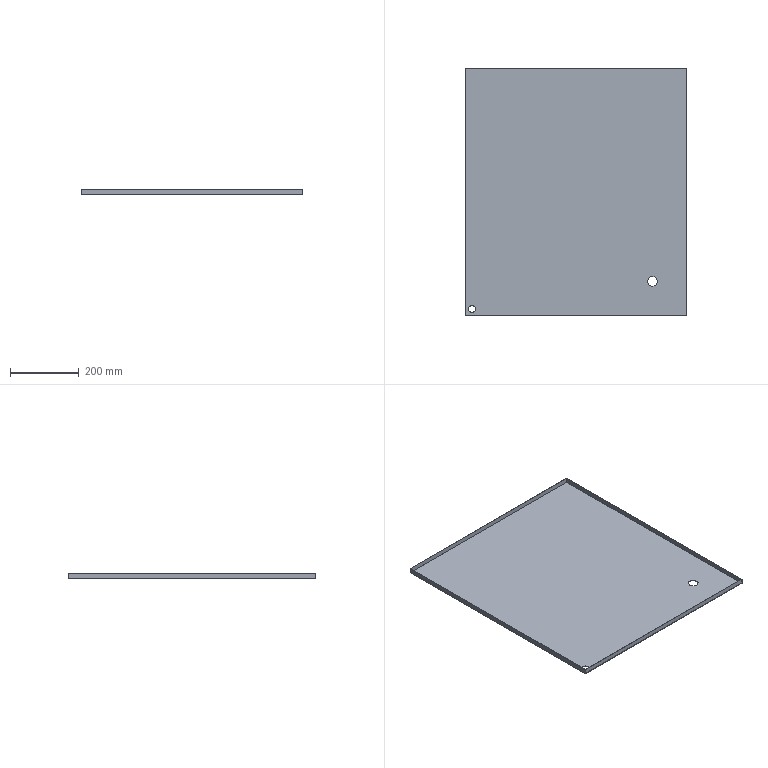Component | SolidWorks | FrameAssembly-1_FrameWeldment-1_RearThinPlate-1 | 1 solid | 15 faces | box 643 x 718 x 15 mm | volume 597890 mm3 | plane 11 | cylinder 4 | commonest cylinder face diameters 20 x2 28 x2
build123d program:
from build123d import *

# Parameters (mm, degrees)
SKETCH1_W                      = 643
SKETCH1_H                      = 718
BOSS_EXTRUDE1_DEPTH            = 15
SKETCH2_W                      = 640.6
SKETCH2_H                      = 715.6
CUT_EXTRUDE1_DEPTH             = 13.8
M24_CLEARANCE_HOLE_1_D         = 28
M24_CLEARANCE_HOLE_1_DEPTH     = 15
F_20_0_20_DIAMETER_HOLE1_D     = 20
F_20_0_20_DIAMETER_HOLE1_DEPTH = 15


with BuildPart() as part:
    # Sketch1 → Boss-Extrude1 (new body)
    with BuildSketch(Plane(origin=(0, 0, 0), x_dir=(-1, 0, 0), z_dir=(0, 0, -1))):
        Rectangle(SKETCH1_W, SKETCH1_H)
    extrude(amount=-BOSS_EXTRUDE1_DEPTH)

    # Sketch2 → Cut-Extrude1 (cut)
    with BuildSketch(Plane(origin=(0, 0, 0), x_dir=(-1, 0, 0), z_dir=(0, 0, -1))):
        Rectangle(SKETCH2_W, SKETCH2_H)
    extrude(amount=-CUT_EXTRUDE1_DEPTH, mode=Mode.SUBTRACT)

    # M24 Clearance Hole 1
    with Locations(Plane.XY.offset(15)):
        with Locations((-221.5, -259)):
            Hole(M24_CLEARANCE_HOLE_1_D / 2, depth=M24_CLEARANCE_HOLE_1_DEPTH)

    # 20.0 _20_ Diameter Hole1
    with Locations(Plane.XY.offset(15)):
        with Locations((301.5, -339)):
            Hole(F_20_0_20_DIAMETER_HOLE1_D / 2, depth=F_20_0_20_DIAMETER_HOLE1_DEPTH)


solid = part.part

# Placed as in the assembly
solid = solid.moved(Location((-298.746, -38.627, -351.5), (-180, 0, 180)))
STEP:
#1=CARTESIAN_POINT('',(-24.025,-14.867,-14.382));
#2=VERTEX_POINT('',#1);
#3=CARTESIAN_POINT('',(-23.238,-14.867,-14.382));
#4=VERTEX_POINT('',#3);
#5=CARTESIAN_POINT('',(-23.632,-14.867,-14.382));
#6=DIRECTION('',(0.,0.,1.));
#7=DIRECTION('',(1.,0.,0.));
#8=AXIS2_PLACEMENT_3D('',#5,#6,#7);
#9=CIRCLE('',#8,0.3937);
#10=EDGE_CURVE('',#2,#4,#9,.T.);
#11=ORIENTED_EDGE('',*,*,#10,.T.);
#12=CARTESIAN_POINT('',(-23.238,-14.867,-14.429));
#13=VERTEX_POINT('',#12);
#14=CARTESIAN_POINT('',(-23.238,-14.867,-14.429));
#15=DIRECTION('',(-0.,-0.,-1.));
#16=VECTOR('',#15,39.37);
#17=LINE('',#14,#16);
#18=EDGE_CURVE('',#4,#13,#17,.T.);
#19=ORIENTED_EDGE('',*,*,#18,.T.);
#20=CARTESIAN_POINT('',(-24.025,-14.867,-14.429));
#21=VERTEX_POINT('',#20);
#22=CARTESIAN_POINT('',(-23.632,-14.867,-14.429));
#23=DIRECTION('',(-0.,-0.,-1.));
#24=DIRECTION('',(-1.,0.,0.));
#25=AXIS2_PLACEMENT_3D('',#22,#23,#24);
#26=CIRCLE('',#25,0.3937);
#27=EDGE_CURVE('',#13,#21,#26,.T.);
#28=ORIENTED_EDGE('',*,*,#27,.T.);
#29=CARTESIAN_POINT('',(-24.025,-14.867,-14.429));
#30=DIRECTION('',(-0.,-0.,-1.));
#31=VECTOR('',#30,39.37);
#32=LINE('',#29,#31);
#33=EDGE_CURVE('',#2,#21,#32,.T.);
#34=ORIENTED_EDGE('',*,*,#33,.F.);
#35=EDGE_LOOP('',(#11,#19,#28,#34));
#36=FACE_OUTER_BOUND('',#35,.T.);
#37=CARTESIAN_POINT('',(-23.632,-14.867,-14.429));
#38=DIRECTION('',(-0.,-0.,-1.));
#39=DIRECTION('',(-1.,0.,0.));
#40=AXIS2_PLACEMENT_3D('',#37,#38,#39);
#41=CYLINDRICAL_SURFACE('',#40,0.3937);
#42=ADVANCED_FACE('',(#36),#41,.F.);
#43=CARTESIAN_POINT('',(-3.592,-11.718,-14.382));
#44=VERTEX_POINT('',#43);
#45=CARTESIAN_POINT('',(-2.49,-11.718,-14.382));
#46=VERTEX_POINT('',#45);
#47=CARTESIAN_POINT('',(-3.041,-11.718,-14.382));
#48=DIRECTION('',(0.,0.,1.));
#49=DIRECTION('',(1.,0.,0.));
#50=AXIS2_PLACEMENT_3D('',#47,#48,#49);
#51=CIRCLE('',#50,0.5512);
#52=EDGE_CURVE('',#44,#46,#51,.T.);
#53=ORIENTED_EDGE('',*,*,#52,.T.);
#54=CARTESIAN_POINT('',(-2.49,-11.718,-14.429));
#55=VERTEX_POINT('',#54);
#56=CARTESIAN_POINT('',(-2.49,-11.718,-14.429));
#57=DIRECTION('',(-0.,-0.,-1.));
#58=VECTOR('',#57,39.37);
#59=LINE('',#56,#58);
#60=EDGE_CURVE('',#46,#55,#59,.T.);
#61=ORIENTED_EDGE('',*,*,#60,.T.);
#62=CARTESIAN_POINT('',(-3.592,-11.718,-14.429));
#63=VERTEX_POINT('',#62);
#64=CARTESIAN_POINT('',(-3.041,-11.718,-14.429));
#65=DIRECTION('',(-0.,-0.,-1.));
#66=DIRECTION('',(-1.,0.,0.));
#67=AXIS2_PLACEMENT_3D('',#64,#65,#66);
#68=CIRCLE('',#67,0.5512);
#69=EDGE_CURVE('',#55,#63,#68,.T.);
#70=ORIENTED_EDGE('',*,*,#69,.T.);
#71=CARTESIAN_POINT('',(-3.592,-11.718,-14.429));
#72=DIRECTION('',(-0.,-0.,-1.));
#73=VECTOR('',#72,39.37);
#74=LINE('',#71,#73);
#75=EDGE_CURVE('',#44,#63,#74,.T.);
#76=ORIENTED_EDGE('',*,*,#75,.F.);
#77=EDGE_LOOP('',(#53,#61,#70,#76));
#78=FACE_OUTER_BOUND('',#77,.T.);
#79=CARTESIAN_POINT('',(-3.041,-11.718,-14.429));
#80=DIRECTION('',(-0.,-0.,-1.));
#81=DIRECTION('',(-1.,0.,0.));
#82=AXIS2_PLACEMENT_3D('',#79,#80,#81);
#83=CYLINDRICAL_SURFACE('',#82,0.5512);
#84=ADVANCED_FACE('',(#78),#83,.F.);
#85=CARTESIAN_POINT('',(-24.419,-15.655,-13.839));
#86=VERTEX_POINT('',#85);
#87=CARTESIAN_POINT('',(0.8958,-15.655,-13.839));
#88=VERTEX_POINT('',#87);
#89=CARTESIAN_POINT('',(-24.419,-15.655,-13.839));
#90=DIRECTION('',(1.,0.,-0.));
#91=VECTOR('',#90,39.37);
#92=LINE('',#89,#91);
#93=EDGE_CURVE('',#86,#88,#92,.T.);
#94=ORIENTED_EDGE('',*,*,#93,.F.);
#95=CARTESIAN_POINT('',(-24.419,-15.655,-14.429));
#96=VERTEX_POINT('',#95);
#97=CARTESIAN_POINT('',(-24.419,-15.655,-14.429));
#98=DIRECTION('',(0.,0.,1.));
#99=VECTOR('',#98,39.37);
#100=LINE('',#97,#99);
#101=EDGE_CURVE('',#96,#86,#100,.T.);
#102=ORIENTED_EDGE('',*,*,#101,.F.);
#103=CARTESIAN_POINT('',(0.8958,-15.655,-14.429));
#104=VERTEX_POINT('',#103);
#105=CARTESIAN_POINT('',(-24.419,-15.655,-14.429));
#106=DIRECTION('',(1.,0.,-0.));
#107=VECTOR('',#106,39.37);
#108=LINE('',#105,#107);
#109=EDGE_CURVE('',#96,#104,#108,.T.);
#110=ORIENTED_EDGE('',*,*,#109,.T.);
#111=CARTESIAN_POINT('',(0.8958,-15.655,-14.429));
#112=DIRECTION('',(0.,0.,1.));
#113=VECTOR('',#112,39.37);
#114=LINE('',#111,#113);
#115=EDGE_CURVE('',#104,#88,#114,.T.);
#116=ORIENTED_EDGE('',*,*,#115,.T.);
#117=EDGE_LOOP('',(#94,#102,#110,#116));
#118=FACE_OUTER_BOUND('',#117,.T.);
#119=CARTESIAN_POINT('',(-24.419,-15.655,-14.429));
#120=DIRECTION('',(0.,-1.,0.));
#121=DIRECTION('',(0.,0.,1.));
#122=AXIS2_PLACEMENT_3D('',#119,#120,#121);
#123=PLANE('',#122);
#124=ADVANCED_FACE('',(#118),#123,.T.);
#125=CARTESIAN_POINT('',(-24.419,12.613,-13.839));
#126=VERTEX_POINT('',#125);
#127=CARTESIAN_POINT('',(-24.419,12.613,-13.839));
#128=DIRECTION('',(0.,-1.,0.));
#129=VECTOR('',#128,39.37);
#130=LINE('',#127,#129);
#131=EDGE_CURVE('',#126,#86,#130,.T.);
#132=ORIENTED_EDGE('',*,*,#131,.F.);
#133=CARTESIAN_POINT('',(-24.419,12.613,-14.429));
#134=VERTEX_POINT('',#133);
#135=CARTESIAN_POINT('',(-24.419,12.613,-14.429));
#136=DIRECTION('',(0.,0.,1.));
#137=VECTOR('',#136,39.37);
#138=LINE('',#135,#137);
#139=EDGE_CURVE('',#134,#126,#138,.T.);
#140=ORIENTED_EDGE('',*,*,#139,.F.);
#141=CARTESIAN_POINT('',(-24.419,12.613,-14.429));
#142=DIRECTION('',(0.,-1.,0.));
#143=VECTOR('',#142,39.37);
#144=LINE('',#141,#143);
#145=EDGE_CURVE('',#134,#96,#144,.T.);
#146=ORIENTED_EDGE('',*,*,#145,.T.);
#147=ORIENTED_EDGE('',*,*,#101,.T.);
#148=EDGE_LOOP('',(#132,#140,#146,#147));
#149=FACE_OUTER_BOUND('',#148,.T.);
#150=CARTESIAN_POINT('',(-24.419,12.613,-14.429));
#151=DIRECTION('',(-1.,-0.,0.));
#152=DIRECTION('',(0.,0.,1.));
#153=AXIS2_PLACEMENT_3D('',#150,#151,#152);
#154=PLANE('',#153);
#155=ADVANCED_FACE('',(#149),#154,.T.);
#156=CARTESIAN_POINT('',(0.8958,12.613,-13.839));
#157=VERTEX_POINT('',#156);
#158=CARTESIAN_POINT('',(0.8958,12.613,-13.839));
#159=DIRECTION('',(-1.,-0.,0.));
#160=VECTOR('',#159,39.37);
#161=LINE('',#158,#160);
#162=EDGE_CURVE('',#157,#126,#161,.T.);
#163=ORIENTED_EDGE('',*,*,#162,.F.);
#164=CARTESIAN_POINT('',(0.8958,12.613,-14.429));
#165=VERTEX_POINT('',#164);
#166=CARTESIAN_POINT('',(0.8958,12.613,-14.429));
#167=DIRECTION('',(0.,0.,1.));
#168=VECTOR('',#167,39.37);
#169=LINE('',#166,#168);
#170=EDGE_CURVE('',#165,#157,#169,.T.);
#171=ORIENTED_EDGE('',*,*,#170,.F.);
#172=CARTESIAN_POINT('',(0.8958,12.613,-14.429));
#173=DIRECTION('',(-1.,-0.,0.));
#174=VECTOR('',#173,39.37);
#175=LINE('',#172,#174);
#176=EDGE_CURVE('',#165,#134,#175,.T.);
#177=ORIENTED_EDGE('',*,*,#176,.T.);
#178=ORIENTED_EDGE('',*,*,#139,.T.);
#179=EDGE_LOOP('',(#163,#171,#177,#178));
#180=FACE_OUTER_BOUND('',#179,.T.);
#181=CARTESIAN_POINT('',(0.8958,12.613,-14.429));
#182=DIRECTION('',(-0.,1.,-0.));
#183=DIRECTION('',(-0.,-0.,-1.));
#184=AXIS2_PLACEMENT_3D('',#181,#182,#183);
#185=PLANE('',#184);
#186=ADVANCED_FACE('',(#180),#185,.T.);
#187=CARTESIAN_POINT('',(0.8958,-15.655,-13.839));
#188=DIRECTION('',(-0.,1.,-0.));
#189=VECTOR('',#188,39.37);
#190=LINE('',#187,#189);
#191=EDGE_CURVE('',#88,#157,#190,.T.);
#192=ORIENTED_EDGE('',*,*,#191,.F.);
#193=ORIENTED_EDGE('',*,*,#115,.F.);
#194=CARTESIAN_POINT('',(0.8958,-15.655,-14.429));
#195=DIRECTION('',(-0.,1.,-0.));
#196=VECTOR('',#195,39.37);
#197=LINE('',#194,#196);
#198=EDGE_CURVE('',#104,#165,#197,.T.);
#199=ORIENTED_EDGE('',*,*,#198,.T.);
#200=ORIENTED_EDGE('',*,*,#170,.T.);
#201=EDGE_LOOP('',(#192,#193,#199,#200));
#202=FACE_OUTER_BOUND('',#201,.T.);
#203=CARTESIAN_POINT('',(0.8958,-15.655,-14.429));
#204=DIRECTION('',(1.,0.,-0.));
#205=DIRECTION('',(-0.,-0.,-1.));
#206=AXIS2_PLACEMENT_3D('',#203,#204,#205);
#207=PLANE('',#206);
#208=ADVANCED_FACE('',(#202),#207,.T.);
#209=CARTESIAN_POINT('',(-23.632,-14.867,-14.429));
#210=DIRECTION('',(-0.,-0.,-1.));
#211=DIRECTION('',(-1.,0.,0.));
#212=AXIS2_PLACEMENT_3D('',#209,#210,#211);
#213=CIRCLE('',#212,0.3937);
#214=EDGE_CURVE('',#21,#13,#213,.T.);
#215=ORIENTED_EDGE('',*,*,#214,.F.);
#216=ORIENTED_EDGE('',*,*,#27,.F.);
#217=EDGE_LOOP('',(#215,#216));
#218=FACE_BOUND('',#217,.T.);
#219=CARTESIAN_POINT('',(-3.041,-11.718,-14.429));
#220=DIRECTION('',(-0.,-0.,-1.));
#221=DIRECTION('',(-1.,0.,0.));
#222=AXIS2_PLACEMENT_3D('',#219,#220,#221);
#223=CIRCLE('',#222,0.5512);
#224=EDGE_CURVE('',#63,#55,#223,.T.);
#225=ORIENTED_EDGE('',*,*,#224,.F.);
#226=ORIENTED_EDGE('',*,*,#69,.F.);
#227=EDGE_LOOP('',(#225,#226));
#228=FACE_BOUND('',#227,.T.);
#229=ORIENTED_EDGE('',*,*,#109,.F.);
#230=ORIENTED_EDGE('',*,*,#145,.F.);
#231=ORIENTED_EDGE('',*,*,#176,.F.);
#232=ORIENTED_EDGE('',*,*,#198,.F.);
#233=EDGE_LOOP('',(#229,#230,#231,#232));
#234=FACE_OUTER_BOUND('',#233,.T.);
#235=CARTESIAN_POINT('',(-11.762,-1.521,-14.429));
#236=DIRECTION('',(0.,0.,1.));
#237=DIRECTION('',(1.,0.,-0.));
#238=AXIS2_PLACEMENT_3D('',#235,#236,#237);
#239=PLANE('',#238);
#240=ADVANCED_FACE('',(#218,#228,#234),#239,.F.);
#241=CARTESIAN_POINT('',(-24.372,12.566,-13.839));
#242=VERTEX_POINT('',#241);
#243=CARTESIAN_POINT('',(-24.372,-15.607,-13.839));
#244=VERTEX_POINT('',#243);
#245=CARTESIAN_POINT('',(-24.372,12.566,-13.839));
#246=DIRECTION('',(0.,-1.,0.));
#247=VECTOR('',#246,39.37);
#248=LINE('',#245,#247);
#249=EDGE_CURVE('',#242,#244,#248,.T.);
#250=ORIENTED_EDGE('',*,*,#249,.F.);
#251=CARTESIAN_POINT('',(0.8486,12.566,-13.839));
#252=VERTEX_POINT('',#251);
#253=CARTESIAN_POINT('',(0.8486,12.566,-13.839));
#254=DIRECTION('',(-1.,-0.,0.));
#255=VECTOR('',#254,39.37);
#256=LINE('',#253,#255);
#257=EDGE_CURVE('',#252,#242,#256,.T.);
#258=ORIENTED_EDGE('',*,*,#257,.F.);
#259=CARTESIAN_POINT('',(0.8486,-15.607,-13.839));
#260=VERTEX_POINT('',#259);
#261=CARTESIAN_POINT('',(0.8486,-15.607,-13.839));
#262=DIRECTION('',(-0.,1.,-0.));
#263=VECTOR('',#262,39.37);
#264=LINE('',#261,#263);
#265=EDGE_CURVE('',#260,#252,#264,.T.);
#266=ORIENTED_EDGE('',*,*,#265,.F.);
#267=CARTESIAN_POINT('',(-24.372,-15.607,-13.839));
#268=DIRECTION('',(1.,0.,-0.));
#269=VECTOR('',#268,39.37);
#270=LINE('',#267,#269);
#271=EDGE_CURVE('',#244,#260,#270,.T.);
#272=ORIENTED_EDGE('',*,*,#271,.F.);
#273=EDGE_LOOP('',(#250,#258,#266,#272));
#274=FACE_BOUND('',#273,.T.);
#275=ORIENTED_EDGE('',*,*,#93,.T.);
#276=ORIENTED_EDGE('',*,*,#191,.T.);
#277=ORIENTED_EDGE('',*,*,#162,.T.);
#278=ORIENTED_EDGE('',*,*,#131,.T.);
#279=EDGE_LOOP('',(#275,#276,#277,#278));
#280=FACE_OUTER_BOUND('',#279,.T.);
#281=CARTESIAN_POINT('',(-11.762,-1.521,-13.839));
#282=DIRECTION('',(0.,0.,1.));
#283=DIRECTION('',(1.,0.,-0.));
#284=AXIS2_PLACEMENT_3D('',#281,#282,#283);
#285=PLANE('',#284);
#286=ADVANCED_FACE('',(#274,#280),#285,.T.);
#287=ORIENTED_EDGE('',*,*,#249,.T.);
#288=CARTESIAN_POINT('',(-24.372,-15.607,-14.382));
#289=VERTEX_POINT('',#288);
#290=CARTESIAN_POINT('',(-24.372,-15.607,-14.382));
#291=DIRECTION('',(0.,0.,1.));
#292=VECTOR('',#291,39.37);
#293=LINE('',#290,#292);
#294=EDGE_CURVE('',#289,#244,#293,.T.);
#295=ORIENTED_EDGE('',*,*,#294,.F.);
#296=CARTESIAN_POINT('',(-24.372,12.566,-14.382));
#297=VERTEX_POINT('',#296);
#298=CARTESIAN_POINT('',(-24.372,12.566,-14.382));
#299=DIRECTION('',(0.,-1.,0.));
#300=VECTOR('',#299,39.37);
#301=LINE('',#298,#300);
#302=EDGE_CURVE('',#297,#289,#301,.T.);
#303=ORIENTED_EDGE('',*,*,#302,.F.);
#304=CARTESIAN_POINT('',(-24.372,12.566,-14.382));
#305=DIRECTION('',(0.,0.,1.));
#306=VECTOR('',#305,39.37);
#307=LINE('',#304,#306);
#308=EDGE_CURVE('',#297,#242,#307,.T.);
#309=ORIENTED_EDGE('',*,*,#308,.T.);
#310=EDGE_LOOP('',(#287,#295,#303,#309));
#311=FACE_OUTER_BOUND('',#310,.T.);
#312=CARTESIAN_POINT('',(-24.372,12.566,-14.382));
#313=DIRECTION('',(-1.,-0.,0.));
#314=DIRECTION('',(-0.,1.,-0.));
#315=AXIS2_PLACEMENT_3D('',#312,#313,#314);
#316=PLANE('',#315);
#317=ADVANCED_FACE('',(#311),#316,.F.);
#318=ORIENTED_EDGE('',*,*,#257,.T.);
#319=ORIENTED_EDGE('',*,*,#308,.F.);
#320=CARTESIAN_POINT('',(0.8486,12.566,-14.382));
#321=VERTEX_POINT('',#320);
#322=CARTESIAN_POINT('',(0.8486,12.566,-14.382));
#323=DIRECTION('',(-1.,-0.,0.));
#324=VECTOR('',#323,39.37);
#325=LINE('',#322,#324);
#326=EDGE_CURVE('',#321,#297,#325,.T.);
#327=ORIENTED_EDGE('',*,*,#326,.F.);
#328=CARTESIAN_POINT('',(0.8486,12.566,-14.382));
#329=DIRECTION('',(0.,0.,1.));
#330=VECTOR('',#329,39.37);
#331=LINE('',#328,#330);
#332=EDGE_CURVE('',#321,#252,#331,.T.);
#333=ORIENTED_EDGE('',*,*,#332,.T.);
#334=EDGE_LOOP('',(#318,#319,#327,#333));
#335=FACE_OUTER_BOUND('',#334,.T.);
#336=CARTESIAN_POINT('',(0.8486,12.566,-14.382));
#337=DIRECTION('',(-0.,1.,-0.));
#338=DIRECTION('',(-0.,-0.,-1.));
#339=AXIS2_PLACEMENT_3D('',#336,#337,#338);
#340=PLANE('',#339);
#341=ADVANCED_FACE('',(#335),#340,.F.);
#342=ORIENTED_EDGE('',*,*,#265,.T.);
#343=ORIENTED_EDGE('',*,*,#332,.F.);
#344=CARTESIAN_POINT('',(0.8486,-15.607,-14.382));
#345=VERTEX_POINT('',#344);
#346=CARTESIAN_POINT('',(0.8486,-15.607,-14.382));
#347=DIRECTION('',(-0.,1.,-0.));
#348=VECTOR('',#347,39.37);
#349=LINE('',#346,#348);
#350=EDGE_CURVE('',#345,#321,#349,.T.);
#351=ORIENTED_EDGE('',*,*,#350,.F.);
#352=CARTESIAN_POINT('',(0.8486,-15.607,-14.382));
#353=DIRECTION('',(0.,0.,1.));
#354=VECTOR('',#353,39.37);
#355=LINE('',#352,#354);
#356=EDGE_CURVE('',#345,#260,#355,.T.);
#357=ORIENTED_EDGE('',*,*,#356,.T.);
#358=EDGE_LOOP('',(#342,#343,#351,#357));
#359=FACE_OUTER_BOUND('',#358,.T.);
#360=CARTESIAN_POINT('',(0.8486,-15.607,-14.382));
#361=DIRECTION('',(1.,0.,-0.));
#362=DIRECTION('',(0.,-1.,0.));
#363=AXIS2_PLACEMENT_3D('',#360,#361,#362);
#364=PLANE('',#363);
#365=ADVANCED_FACE('',(#359),#364,.F.);
#366=ORIENTED_EDGE('',*,*,#271,.T.);
#367=ORIENTED_EDGE('',*,*,#356,.F.);
#368=CARTESIAN_POINT('',(-24.372,-15.607,-14.382));
#369=DIRECTION('',(1.,0.,-0.));
#370=VECTOR('',#369,39.37);
#371=LINE('',#368,#370);
#372=EDGE_CURVE('',#289,#345,#371,.T.);
#373=ORIENTED_EDGE('',*,*,#372,.F.);
#374=ORIENTED_EDGE('',*,*,#294,.T.);
#375=EDGE_LOOP('',(#366,#367,#373,#374));
#376=FACE_OUTER_BOUND('',#375,.T.);
#377=CARTESIAN_POINT('',(-24.372,-15.607,-14.382));
#378=DIRECTION('',(0.,-1.,0.));
#379=DIRECTION('',(0.,0.,1.));
#380=AXIS2_PLACEMENT_3D('',#377,#378,#379);
#381=PLANE('',#380);
#382=ADVANCED_FACE('',(#376),#381,.F.);
#383=ORIENTED_EDGE('',*,*,#10,.F.);
#384=CARTESIAN_POINT('',(-23.632,-14.867,-14.382));
#385=DIRECTION('',(0.,0.,1.));
#386=DIRECTION('',(1.,0.,0.));
#387=AXIS2_PLACEMENT_3D('',#384,#385,#386);
#388=CIRCLE('',#387,0.3937);
#389=EDGE_CURVE('',#4,#2,#388,.T.);
#390=ORIENTED_EDGE('',*,*,#389,.F.);
#391=EDGE_LOOP('',(#383,#390));
#392=FACE_BOUND('',#391,.T.);
#393=ORIENTED_EDGE('',*,*,#52,.F.);
#394=CARTESIAN_POINT('',(-3.041,-11.718,-14.382));
#395=DIRECTION('',(0.,0.,1.));
#396=DIRECTION('',(1.,0.,0.));
#397=AXIS2_PLACEMENT_3D('',#394,#395,#396);
#398=CIRCLE('',#397,0.5512);
#399=EDGE_CURVE('',#46,#44,#398,.T.);
#400=ORIENTED_EDGE('',*,*,#399,.F.);
#401=EDGE_LOOP('',(#393,#400));
#402=FACE_BOUND('',#401,.T.);
#403=ORIENTED_EDGE('',*,*,#302,.T.);
#404=ORIENTED_EDGE('',*,*,#372,.T.);
#405=ORIENTED_EDGE('',*,*,#350,.T.);
#406=ORIENTED_EDGE('',*,*,#326,.T.);
#407=EDGE_LOOP('',(#403,#404,#405,#406));
#408=FACE_OUTER_BOUND('',#407,.T.);
#409=CARTESIAN_POINT('',(-11.762,-1.521,-14.382));
#410=DIRECTION('',(0.,0.,1.));
#411=DIRECTION('',(1.,0.,-0.));
#412=AXIS2_PLACEMENT_3D('',#409,#410,#411);
#413=PLANE('',#412);
#414=ADVANCED_FACE('',(#392,#402,#408),#413,.T.);
#415=ORIENTED_EDGE('',*,*,#60,.F.);
#416=ORIENTED_EDGE('',*,*,#399,.T.);
#417=ORIENTED_EDGE('',*,*,#75,.T.);
#418=ORIENTED_EDGE('',*,*,#224,.T.);
#419=EDGE_LOOP('',(#415,#416,#417,#418));
#420=FACE_OUTER_BOUND('',#419,.T.);
#421=CARTESIAN_POINT('',(-3.041,-11.718,-14.429));
#422=DIRECTION('',(-0.,-0.,-1.));
#423=DIRECTION('',(-1.,0.,0.));
#424=AXIS2_PLACEMENT_3D('',#421,#422,#423);
#425=CYLINDRICAL_SURFACE('',#424,0.5512);
#426=ADVANCED_FACE('',(#420),#425,.F.);
#427=ORIENTED_EDGE('',*,*,#18,.F.);
#428=ORIENTED_EDGE('',*,*,#389,.T.);
#429=ORIENTED_EDGE('',*,*,#33,.T.);
#430=ORIENTED_EDGE('',*,*,#214,.T.);
#431=EDGE_LOOP('',(#427,#428,#429,#430));
#432=FACE_OUTER_BOUND('',#431,.T.);
#433=CARTESIAN_POINT('',(-23.632,-14.867,-14.429));
#434=DIRECTION('',(-0.,-0.,-1.));
#435=DIRECTION('',(-1.,0.,0.));
#436=AXIS2_PLACEMENT_3D('',#433,#434,#435);
#437=CYLINDRICAL_SURFACE('',#436,0.3937);
#438=ADVANCED_FACE('',(#432),#437,.F.);
#439=CLOSED_SHELL('',(#42,#84,#124,#155,#186,#208,#240,#286,#317,#341,#365,#382,#414,#426,#438));
#440=MANIFOLD_SOLID_BREP('',#439);
#441=CARTESIAN_POINT('',(0.,0.,0.));
#442=DIRECTION('',(0.,0.,1.));
#443=DIRECTION('',(1.,0.,0.));
#444=AXIS2_PLACEMENT_3D('',#441,#442,#443);
#445=(LENGTH_UNIT()NAMED_UNIT(*)SI_UNIT($,.METRE.));
#446=LENGTH_MEASURE_WITH_UNIT(LENGTH_MEASURE(0.0254),#445);
#447=DIMENSIONAL_EXPONENTS(1.,0.,0.,0.,0.,0.,0.);
#448=(CONVERSION_BASED_UNIT('',#446)LENGTH_UNIT()NAMED_UNIT(#447));
#449=UNCERTAINTY_MEASURE_WITH_UNIT(LENGTH_MEASURE(0.00001),#448,'','');
#450=(NAMED_UNIT(*)PLANE_ANGLE_UNIT()SI_UNIT($,.RADIAN.));
#451=(NAMED_UNIT(*)SI_UNIT($,.STERADIAN.)SOLID_ANGLE_UNIT());
#452=(GEOMETRIC_REPRESENTATION_CONTEXT(3)GLOBAL_UNCERTAINTY_ASSIGNED_CONTEXT((#449))GLOBAL_UNIT_ASSIGNED_CONTEXT((#448,#450,#451))REPRESENTATION_CONTEXT('',''));
#453=ADVANCED_BREP_SHAPE_REPRESENTATION('',(#440,#444),#452);
#454=COLOUR_RGB('',0.7922,0.8196,0.9333);
#455=FILL_AREA_STYLE_COLOUR('',#454);
#456=FILL_AREA_STYLE('',(#455));
#457=SURFACE_STYLE_FILL_AREA(#456);
#458=SURFACE_SIDE_STYLE('',(#457));
#459=SURFACE_STYLE_USAGE(.BOTH.,#458);
#460=PRESENTATION_STYLE_ASSIGNMENT((#459));
#461=STYLED_ITEM('',(#460),#440);
#462=(LENGTH_UNIT()NAMED_UNIT(*)SI_UNIT($,.METRE.));
#463=LENGTH_MEASURE_WITH_UNIT(LENGTH_MEASURE(0.0254),#462);
#464=DIMENSIONAL_EXPONENTS(1.,0.,0.,0.,0.,0.,0.);
#465=(CONVERSION_BASED_UNIT('',#463)LENGTH_UNIT()NAMED_UNIT(#464));
#466=UNCERTAINTY_MEASURE_WITH_UNIT(LENGTH_MEASURE(0.00001),#465,'','');
#467=(NAMED_UNIT(*)PLANE_ANGLE_UNIT()SI_UNIT($,.RADIAN.));
#468=(NAMED_UNIT(*)SI_UNIT($,.STERADIAN.)SOLID_ANGLE_UNIT());
#469=(GEOMETRIC_REPRESENTATION_CONTEXT(3)GLOBAL_UNCERTAINTY_ASSIGNED_CONTEXT((#466))GLOBAL_UNIT_ASSIGNED_CONTEXT((#465,#467,#468))REPRESENTATION_CONTEXT('',''));
#470=MECHANICAL_DESIGN_GEOMETRIC_PRESENTATION_REPRESENTATION('',(#461),#469);
#471=PRESENTATION_LAYER_ASSIGNMENT('','',(#461));